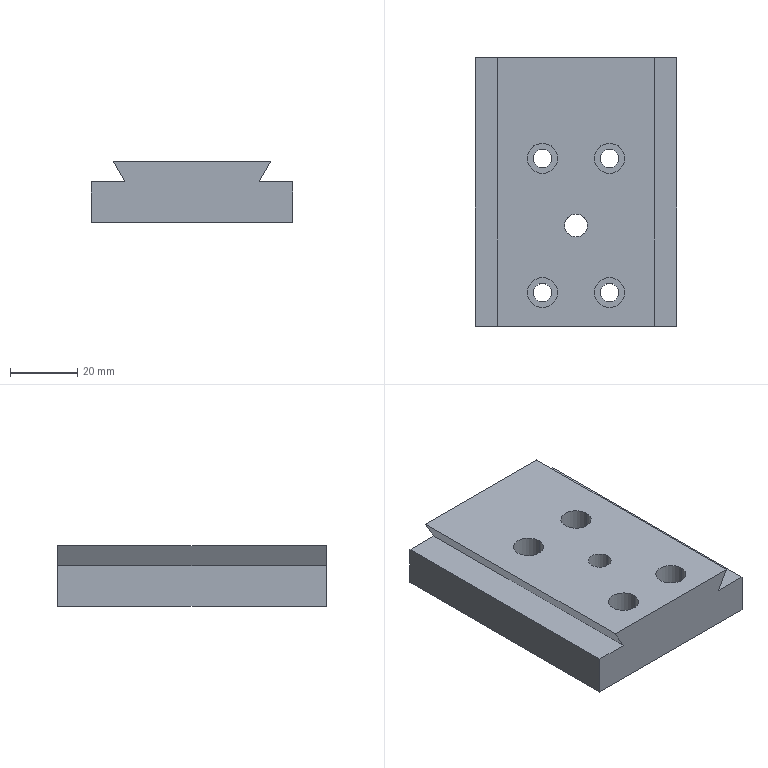Component | SolidWorks | DovetailBase1-1 | 1 solid | 40 faces | box 60 x 80 x 18 mm | volume 74627 mm3 | cylinder 22 | plane 14 | cone 4 | commonest cylinder face diameters 9 x8 5.5 x8 4.2 x4 6.8 x2
build123d program:
from build123d import *

# Parameters (mm, degrees)
SKETCH1_W                                          = 60
SKETCH1_H                                          = 80
BOSS_EXTRUDE1_DEPTH                                = 18
CUT_EXTRUDE1_DEPTH                                 = 84
M8_TAPPED_HOLE1_D                                  = 6.8
HOLE_SIZE_ACCORDING_TO_TYPE_1_OF_HEXAG_D           = 5.5
HOLE_SIZE_ACCORDING_TO_TYPE_1_OF_HEXAG_CBORE_D     = 9
HOLE_SIZE_ACCORDING_TO_TYPE_1_OF_HEXAG_CBORE_DEPTH = 7
M5_TAPPED_HOLE1_D                                  = 4.2
M5_TAPPED_HOLE1_DEPTH                              = 12.4
M5_TAPPED_HOLE1_TIP                                = 1.262


with BuildPart() as part:
    # Sketch1 → Boss-Extrude1 (new body)
    with BuildSketch(Plane.XY):
        Rectangle(SKETCH1_W, SKETCH1_H)
    extrude(amount=BOSS_EXTRUDE1_DEPTH)

    # Sketch2 → Cut-Extrude1 (cut)
    with BuildSketch(Plane(origin=(0, 40, 0), x_dir=(1, 0, 0), z_dir=(0, 1, 0))):
        Polygon((-20, -12), (-30, -12), (-30, -18), (-23.464, -18), align=None)
        Polygon((20, -12), (23.464, -18), (30, -18), (30, -12), align=None)
    extrude(amount=-CUT_EXTRUDE1_DEPTH, mode=Mode.SUBTRACT)

    # M8 Tapped Hole1 (through all)
    with Locations(Plane(origin=(0, -10, 18), x_dir=(1, 0, 0), z_dir=(0, 0, 1))):
        with Locations((0, 0)):
            Hole(M8_TAPPED_HOLE1_D / 2)

    # Hole Size _according to_ Type 1 of Hexag (through all)
    with Locations(Plane(origin=(-10, -30, 18), x_dir=(1, 0, 0), z_dir=(0, 0, 1))):
        with Locations((0, 0), (20, 0), (20, 40), (0, 40)):
            CounterBoreHole(HOLE_SIZE_ACCORDING_TO_TYPE_1_OF_HEXAG_D / 2, HOLE_SIZE_ACCORDING_TO_TYPE_1_OF_HEXAG_CBORE_D / 2, HOLE_SIZE_ACCORDING_TO_TYPE_1_OF_HEXAG_CBORE_DEPTH)

    # M5 Tapped Hole1
    with Locations(Plane(origin=(-10, 40, 7), x_dir=(0, 0, 1), z_dir=(0, 1, 0))):
        with Locations((0, 0), (0, 20)):
            Hole(M5_TAPPED_HOLE1_D / 2, depth=M5_TAPPED_HOLE1_DEPTH)
            with Locations((0, 0, -(M5_TAPPED_HOLE1_DEPTH + M5_TAPPED_HOLE1_TIP / 2))):  # 118° drill point
                Cone(0, M5_TAPPED_HOLE1_D / 2, M5_TAPPED_HOLE1_TIP, mode=Mode.SUBTRACT)


solid = part.part

# Placed as in the assembly
solid = solid.moved(Location((-48.047, -14.04, -9), (0, 0, 0)))